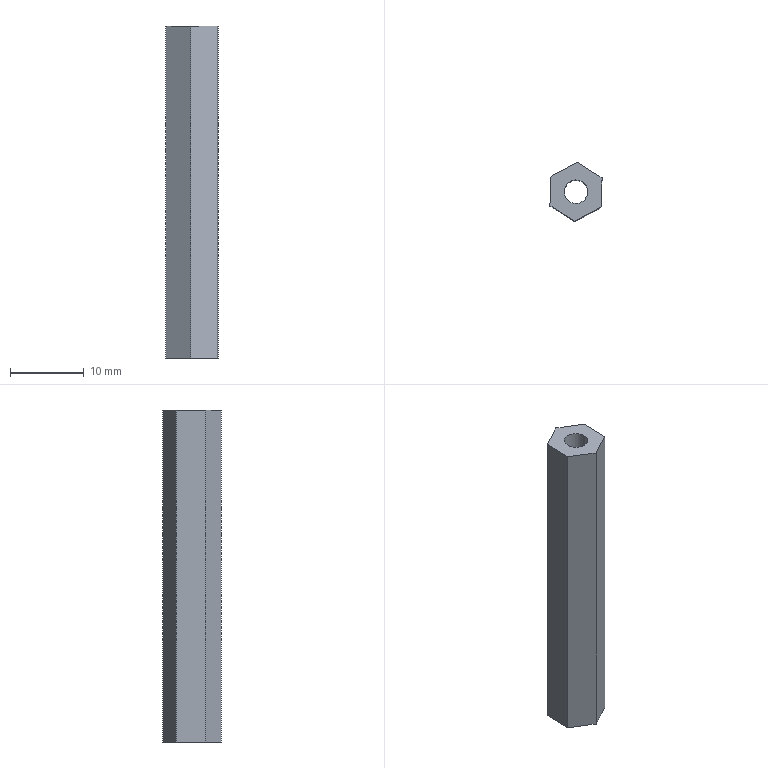Component | SolidWorks | 25CopperPillar-Copy-1 | 1 solid | 10 faces | box 7.07 x 7.99 x 45 mm | volume 1509 mm3 | plane 8 | cylinder 2 | commonest cylinder face diameters 3.2 x2
STEP:
#1=CARTESIAN_POINT('',(1.915,2.002,1.929));
#2=VERTEX_POINT('',#1);
#3=CARTESIAN_POINT('',(2.022,1.935,1.929));
#4=VERTEX_POINT('',#3);
#5=CARTESIAN_POINT('',(1.969,1.969,1.929));
#6=DIRECTION('',(0.,0.,1.));
#7=DIRECTION('',(0.8471,-0.5314,0.));
#8=AXIS2_PLACEMENT_3D('',#5,#6,#7);
#9=CIRCLE('',#8,0.06299);
#10=EDGE_CURVE('',#2,#4,#9,.T.);
#11=ORIENTED_EDGE('',*,*,#10,.T.);
#12=CARTESIAN_POINT('',(2.022,1.935,0.1575));
#13=VERTEX_POINT('',#12);
#14=CARTESIAN_POINT('',(2.022,1.935,1.929));
#15=DIRECTION('',(0.,0.,-1.));
#16=VECTOR('',#15,39.37);
#17=LINE('',#14,#16);
#18=EDGE_CURVE('',#4,#13,#17,.T.);
#19=ORIENTED_EDGE('',*,*,#18,.T.);
#20=CARTESIAN_POINT('',(1.915,2.002,0.1575));
#21=VERTEX_POINT('',#20);
#22=CARTESIAN_POINT('',(1.969,1.969,0.1575));
#23=DIRECTION('',(0.,0.,1.));
#24=DIRECTION('',(0.8471,-0.5314,0.));
#25=AXIS2_PLACEMENT_3D('',#22,#23,#24);
#26=CIRCLE('',#25,0.06299);
#27=EDGE_CURVE('',#21,#13,#26,.T.);
#28=ORIENTED_EDGE('',*,*,#27,.F.);
#29=CARTESIAN_POINT('',(1.915,2.002,1.929));
#30=DIRECTION('',(0.,0.,-1.));
#31=VECTOR('',#30,39.37);
#32=LINE('',#29,#31);
#33=EDGE_CURVE('',#2,#21,#32,.T.);
#34=ORIENTED_EDGE('',*,*,#33,.F.);
#35=EDGE_LOOP('',(#11,#19,#28,#34));
#36=FACE_OUTER_BOUND('',#35,.T.);
#37=CARTESIAN_POINT('',(1.969,1.969,1.929));
#38=DIRECTION('',(0.,0.,-1.));
#39=DIRECTION('',(-0.8471,0.5314,0.));
#40=AXIS2_PLACEMENT_3D('',#37,#38,#39);
#41=CYLINDRICAL_SURFACE('',#40,0.06299);
#42=ADVANCED_FACE('',(#36),#41,.F.);
#43=CARTESIAN_POINT('',(1.963,1.811,1.929));
#44=VERTEX_POINT('',#43);
#45=CARTESIAN_POINT('',(2.102,1.885,1.929));
#46=VERTEX_POINT('',#45);
#47=CARTESIAN_POINT('',(1.963,1.811,1.929));
#48=DIRECTION('',(0.8838,0.4679,0.));
#49=VECTOR('',#48,39.37);
#50=LINE('',#47,#49);
#51=EDGE_CURVE('',#44,#46,#50,.T.);
#52=ORIENTED_EDGE('',*,*,#51,.T.);
#53=CARTESIAN_POINT('',(2.108,2.042,1.929));
#54=VERTEX_POINT('',#53);
#55=CARTESIAN_POINT('',(2.102,1.885,1.929));
#56=DIRECTION('',(0.03664,0.9993,0.));
#57=VECTOR('',#56,39.37);
#58=LINE('',#55,#57);
#59=EDGE_CURVE('',#46,#54,#58,.T.);
#60=ORIENTED_EDGE('',*,*,#59,.T.);
#61=CARTESIAN_POINT('',(1.974,2.126,1.929));
#62=VERTEX_POINT('',#61);
#63=CARTESIAN_POINT('',(2.108,2.042,1.929));
#64=DIRECTION('',(-0.8471,0.5314,0.));
#65=VECTOR('',#64,39.37);
#66=LINE('',#63,#65);
#67=EDGE_CURVE('',#54,#62,#66,.T.);
#68=ORIENTED_EDGE('',*,*,#67,.T.);
#69=CARTESIAN_POINT('',(1.835,2.052,1.929));
#70=VERTEX_POINT('',#69);
#71=CARTESIAN_POINT('',(1.974,2.126,1.929));
#72=DIRECTION('',(-0.8838,-0.4679,0.));
#73=VECTOR('',#72,39.37);
#74=LINE('',#71,#73);
#75=EDGE_CURVE('',#62,#70,#74,.T.);
#76=ORIENTED_EDGE('',*,*,#75,.T.);
#77=CARTESIAN_POINT('',(1.829,1.895,1.929));
#78=VERTEX_POINT('',#77);
#79=CARTESIAN_POINT('',(1.835,2.052,1.929));
#80=DIRECTION('',(-0.03664,-0.9993,0.));
#81=VECTOR('',#80,39.37);
#82=LINE('',#79,#81);
#83=EDGE_CURVE('',#70,#78,#82,.T.);
#84=ORIENTED_EDGE('',*,*,#83,.T.);
#85=CARTESIAN_POINT('',(1.829,1.895,1.929));
#86=DIRECTION('',(0.8471,-0.5314,0.));
#87=VECTOR('',#86,39.37);
#88=LINE('',#85,#87);
#89=EDGE_CURVE('',#78,#44,#88,.T.);
#90=ORIENTED_EDGE('',*,*,#89,.T.);
#91=EDGE_LOOP('',(#52,#60,#68,#76,#84,#90));
#92=FACE_OUTER_BOUND('',#91,.T.);
#93=ORIENTED_EDGE('',*,*,#10,.F.);
#94=CARTESIAN_POINT('',(1.969,1.969,1.929));
#95=DIRECTION('',(0.,0.,1.));
#96=DIRECTION('',(0.8471,-0.5314,0.));
#97=AXIS2_PLACEMENT_3D('',#94,#95,#96);
#98=CIRCLE('',#97,0.06299);
#99=EDGE_CURVE('',#4,#2,#98,.T.);
#100=ORIENTED_EDGE('',*,*,#99,.F.);
#101=EDGE_LOOP('',(#93,#100));
#102=FACE_BOUND('',#101,.T.);
#103=CARTESIAN_POINT('',(1.969,1.969,1.929));
#104=DIRECTION('',(0.,0.,1.));
#105=DIRECTION('',(0.8471,-0.5314,0.));
#106=AXIS2_PLACEMENT_3D('',#103,#104,#105);
#107=PLANE('',#106);
#108=ADVANCED_FACE('',(#92,#102),#107,.T.);
#109=CARTESIAN_POINT('',(1.963,1.811,0.1575));
#110=VERTEX_POINT('',#109);
#111=CARTESIAN_POINT('',(2.102,1.885,0.1575));
#112=VERTEX_POINT('',#111);
#113=CARTESIAN_POINT('',(1.963,1.811,0.1575));
#114=DIRECTION('',(0.8838,0.4679,0.));
#115=VECTOR('',#114,39.37);
#116=LINE('',#113,#115);
#117=EDGE_CURVE('',#110,#112,#116,.T.);
#118=ORIENTED_EDGE('',*,*,#117,.F.);
#119=CARTESIAN_POINT('',(1.829,1.895,0.1575));
#120=VERTEX_POINT('',#119);
#121=CARTESIAN_POINT('',(1.829,1.895,0.1575));
#122=DIRECTION('',(0.8471,-0.5314,0.));
#123=VECTOR('',#122,39.37);
#124=LINE('',#121,#123);
#125=EDGE_CURVE('',#120,#110,#124,.T.);
#126=ORIENTED_EDGE('',*,*,#125,.F.);
#127=CARTESIAN_POINT('',(1.835,2.052,0.1575));
#128=VERTEX_POINT('',#127);
#129=CARTESIAN_POINT('',(1.835,2.052,0.1575));
#130=DIRECTION('',(-0.03664,-0.9993,0.));
#131=VECTOR('',#130,39.37);
#132=LINE('',#129,#131);
#133=EDGE_CURVE('',#128,#120,#132,.T.);
#134=ORIENTED_EDGE('',*,*,#133,.F.);
#135=CARTESIAN_POINT('',(1.974,2.126,0.1575));
#136=VERTEX_POINT('',#135);
#137=CARTESIAN_POINT('',(1.974,2.126,0.1575));
#138=DIRECTION('',(-0.8838,-0.4679,0.));
#139=VECTOR('',#138,39.37);
#140=LINE('',#137,#139);
#141=EDGE_CURVE('',#136,#128,#140,.T.);
#142=ORIENTED_EDGE('',*,*,#141,.F.);
#143=CARTESIAN_POINT('',(2.108,2.042,0.1575));
#144=VERTEX_POINT('',#143);
#145=CARTESIAN_POINT('',(2.108,2.042,0.1575));
#146=DIRECTION('',(-0.8471,0.5314,0.));
#147=VECTOR('',#146,39.37);
#148=LINE('',#145,#147);
#149=EDGE_CURVE('',#144,#136,#148,.T.);
#150=ORIENTED_EDGE('',*,*,#149,.F.);
#151=CARTESIAN_POINT('',(2.102,1.885,0.1575));
#152=DIRECTION('',(0.03664,0.9993,0.));
#153=VECTOR('',#152,39.37);
#154=LINE('',#151,#153);
#155=EDGE_CURVE('',#112,#144,#154,.T.);
#156=ORIENTED_EDGE('',*,*,#155,.F.);
#157=EDGE_LOOP('',(#118,#126,#134,#142,#150,#156));
#158=FACE_OUTER_BOUND('',#157,.T.);
#159=ORIENTED_EDGE('',*,*,#27,.T.);
#160=CARTESIAN_POINT('',(1.969,1.969,0.1575));
#161=DIRECTION('',(0.,0.,1.));
#162=DIRECTION('',(0.8471,-0.5314,0.));
#163=AXIS2_PLACEMENT_3D('',#160,#161,#162);
#164=CIRCLE('',#163,0.06299);
#165=EDGE_CURVE('',#13,#21,#164,.T.);
#166=ORIENTED_EDGE('',*,*,#165,.T.);
#167=EDGE_LOOP('',(#159,#166));
#168=FACE_BOUND('',#167,.T.);
#169=CARTESIAN_POINT('',(1.969,1.969,0.1575));
#170=DIRECTION('',(0.,0.,1.));
#171=DIRECTION('',(0.8471,-0.5314,0.));
#172=AXIS2_PLACEMENT_3D('',#169,#170,#171);
#173=PLANE('',#172);
#174=ADVANCED_FACE('',(#158,#168),#173,.F.);
#175=ORIENTED_EDGE('',*,*,#117,.T.);
#176=CARTESIAN_POINT('',(2.102,1.885,1.929));
#177=DIRECTION('',(0.,0.,-1.));
#178=VECTOR('',#177,39.37);
#179=LINE('',#176,#178);
#180=EDGE_CURVE('',#46,#112,#179,.T.);
#181=ORIENTED_EDGE('',*,*,#180,.F.);
#182=ORIENTED_EDGE('',*,*,#51,.F.);
#183=CARTESIAN_POINT('',(1.963,1.811,1.929));
#184=DIRECTION('',(0.,0.,-1.));
#185=VECTOR('',#184,39.37);
#186=LINE('',#183,#185);
#187=EDGE_CURVE('',#44,#110,#186,.T.);
#188=ORIENTED_EDGE('',*,*,#187,.T.);
#189=EDGE_LOOP('',(#175,#181,#182,#188));
#190=FACE_OUTER_BOUND('',#189,.T.);
#191=CARTESIAN_POINT('',(1.963,1.811,1.929));
#192=DIRECTION('',(-0.4679,0.8838,0.));
#193=DIRECTION('',(-0.8838,-0.4679,0.));
#194=AXIS2_PLACEMENT_3D('',#191,#192,#193);
#195=PLANE('',#194);
#196=ADVANCED_FACE('',(#190),#195,.F.);
#197=ORIENTED_EDGE('',*,*,#155,.T.);
#198=CARTESIAN_POINT('',(2.108,2.042,1.929));
#199=DIRECTION('',(0.,0.,-1.));
#200=VECTOR('',#199,39.37);
#201=LINE('',#198,#200);
#202=EDGE_CURVE('',#54,#144,#201,.T.);
#203=ORIENTED_EDGE('',*,*,#202,.F.);
#204=ORIENTED_EDGE('',*,*,#59,.F.);
#205=ORIENTED_EDGE('',*,*,#180,.T.);
#206=EDGE_LOOP('',(#197,#203,#204,#205));
#207=FACE_OUTER_BOUND('',#206,.T.);
#208=CARTESIAN_POINT('',(2.102,1.885,1.929));
#209=DIRECTION('',(-0.9993,0.03664,0.));
#210=DIRECTION('',(-0.03664,-0.9993,0.));
#211=AXIS2_PLACEMENT_3D('',#208,#209,#210);
#212=PLANE('',#211);
#213=ADVANCED_FACE('',(#207),#212,.F.);
#214=ORIENTED_EDGE('',*,*,#149,.T.);
#215=CARTESIAN_POINT('',(1.974,2.126,1.929));
#216=DIRECTION('',(0.,0.,-1.));
#217=VECTOR('',#216,39.37);
#218=LINE('',#215,#217);
#219=EDGE_CURVE('',#62,#136,#218,.T.);
#220=ORIENTED_EDGE('',*,*,#219,.F.);
#221=ORIENTED_EDGE('',*,*,#67,.F.);
#222=ORIENTED_EDGE('',*,*,#202,.T.);
#223=EDGE_LOOP('',(#214,#220,#221,#222));
#224=FACE_OUTER_BOUND('',#223,.T.);
#225=CARTESIAN_POINT('',(2.108,2.042,1.929));
#226=DIRECTION('',(-0.5314,-0.8471,0.));
#227=DIRECTION('',(0.8471,-0.5314,0.));
#228=AXIS2_PLACEMENT_3D('',#225,#226,#227);
#229=PLANE('',#228);
#230=ADVANCED_FACE('',(#224),#229,.F.);
#231=ORIENTED_EDGE('',*,*,#141,.T.);
#232=CARTESIAN_POINT('',(1.835,2.052,1.929));
#233=DIRECTION('',(0.,0.,-1.));
#234=VECTOR('',#233,39.37);
#235=LINE('',#232,#234);
#236=EDGE_CURVE('',#70,#128,#235,.T.);
#237=ORIENTED_EDGE('',*,*,#236,.F.);
#238=ORIENTED_EDGE('',*,*,#75,.F.);
#239=ORIENTED_EDGE('',*,*,#219,.T.);
#240=EDGE_LOOP('',(#231,#237,#238,#239));
#241=FACE_OUTER_BOUND('',#240,.T.);
#242=CARTESIAN_POINT('',(1.974,2.126,1.929));
#243=DIRECTION('',(0.4679,-0.8838,0.));
#244=DIRECTION('',(0.8838,0.4679,0.));
#245=AXIS2_PLACEMENT_3D('',#242,#243,#244);
#246=PLANE('',#245);
#247=ADVANCED_FACE('',(#241),#246,.F.);
#248=ORIENTED_EDGE('',*,*,#133,.T.);
#249=CARTESIAN_POINT('',(1.829,1.895,1.929));
#250=DIRECTION('',(0.,0.,-1.));
#251=VECTOR('',#250,39.37);
#252=LINE('',#249,#251);
#253=EDGE_CURVE('',#78,#120,#252,.T.);
#254=ORIENTED_EDGE('',*,*,#253,.F.);
#255=ORIENTED_EDGE('',*,*,#83,.F.);
#256=ORIENTED_EDGE('',*,*,#236,.T.);
#257=EDGE_LOOP('',(#248,#254,#255,#256));
#258=FACE_OUTER_BOUND('',#257,.T.);
#259=CARTESIAN_POINT('',(1.835,2.052,1.929));
#260=DIRECTION('',(0.9993,-0.03664,0.));
#261=DIRECTION('',(0.03664,0.9993,0.));
#262=AXIS2_PLACEMENT_3D('',#259,#260,#261);
#263=PLANE('',#262);
#264=ADVANCED_FACE('',(#258),#263,.F.);
#265=ORIENTED_EDGE('',*,*,#125,.T.);
#266=ORIENTED_EDGE('',*,*,#187,.F.);
#267=ORIENTED_EDGE('',*,*,#89,.F.);
#268=ORIENTED_EDGE('',*,*,#253,.T.);
#269=EDGE_LOOP('',(#265,#266,#267,#268));
#270=FACE_OUTER_BOUND('',#269,.T.);
#271=CARTESIAN_POINT('',(1.829,1.895,1.929));
#272=DIRECTION('',(0.5314,0.8471,0.));
#273=DIRECTION('',(-0.8471,0.5314,0.));
#274=AXIS2_PLACEMENT_3D('',#271,#272,#273);
#275=PLANE('',#274);
#276=ADVANCED_FACE('',(#270),#275,.F.);
#277=ORIENTED_EDGE('',*,*,#18,.F.);
#278=ORIENTED_EDGE('',*,*,#99,.T.);
#279=ORIENTED_EDGE('',*,*,#33,.T.);
#280=ORIENTED_EDGE('',*,*,#165,.F.);
#281=EDGE_LOOP('',(#277,#278,#279,#280));
#282=FACE_OUTER_BOUND('',#281,.T.);
#283=CARTESIAN_POINT('',(1.969,1.969,1.929));
#284=DIRECTION('',(0.,0.,-1.));
#285=DIRECTION('',(-0.8471,0.5314,0.));
#286=AXIS2_PLACEMENT_3D('',#283,#284,#285);
#287=CYLINDRICAL_SURFACE('',#286,0.06299);
#288=ADVANCED_FACE('',(#282),#287,.F.);
#289=CLOSED_SHELL('',(#42,#108,#174,#196,#213,#230,#247,#264,#276,#288));
#290=MANIFOLD_SOLID_BREP('',#289);
#291=CARTESIAN_POINT('',(0.,0.,0.));
#292=DIRECTION('',(0.,0.,1.));
#293=DIRECTION('',(1.,0.,0.));
#294=AXIS2_PLACEMENT_3D('',#291,#292,#293);
#295=(LENGTH_UNIT()NAMED_UNIT(*)SI_UNIT($,.METRE.));
#296=LENGTH_MEASURE_WITH_UNIT(LENGTH_MEASURE(0.0254),#295);
#297=DIMENSIONAL_EXPONENTS(1.,0.,0.,0.,0.,0.,0.);
#298=(CONVERSION_BASED_UNIT('',#296)LENGTH_UNIT()NAMED_UNIT(#297));
#299=UNCERTAINTY_MEASURE_WITH_UNIT(LENGTH_MEASURE(0.00001),#298,'','');
#300=(NAMED_UNIT(*)PLANE_ANGLE_UNIT()SI_UNIT($,.RADIAN.));
#301=(NAMED_UNIT(*)SI_UNIT($,.STERADIAN.)SOLID_ANGLE_UNIT());
#302=(GEOMETRIC_REPRESENTATION_CONTEXT(3)GLOBAL_UNCERTAINTY_ASSIGNED_CONTEXT((#299))GLOBAL_UNIT_ASSIGNED_CONTEXT((#298,#300,#301))REPRESENTATION_CONTEXT('',''));
#303=ADVANCED_BREP_SHAPE_REPRESENTATION('',(#290,#294),#302);
#304=COLOUR_RGB('',0.7922,0.8196,0.9333);
#305=FILL_AREA_STYLE_COLOUR('',#304);
#306=FILL_AREA_STYLE('',(#305));
#307=SURFACE_STYLE_FILL_AREA(#306);
#308=SURFACE_SIDE_STYLE('',(#307));
#309=SURFACE_STYLE_USAGE(.BOTH.,#308);
#310=PRESENTATION_STYLE_ASSIGNMENT((#309));
#311=STYLED_ITEM('',(#310),#290);
#312=(LENGTH_UNIT()NAMED_UNIT(*)SI_UNIT($,.METRE.));
#313=LENGTH_MEASURE_WITH_UNIT(LENGTH_MEASURE(0.0254),#312);
#314=DIMENSIONAL_EXPONENTS(1.,0.,0.,0.,0.,0.,0.);
#315=(CONVERSION_BASED_UNIT('',#313)LENGTH_UNIT()NAMED_UNIT(#314));
#316=UNCERTAINTY_MEASURE_WITH_UNIT(LENGTH_MEASURE(0.00001),#315,'','');
#317=(NAMED_UNIT(*)PLANE_ANGLE_UNIT()SI_UNIT($,.RADIAN.));
#318=(NAMED_UNIT(*)SI_UNIT($,.STERADIAN.)SOLID_ANGLE_UNIT());
#319=(GEOMETRIC_REPRESENTATION_CONTEXT(3)GLOBAL_UNCERTAINTY_ASSIGNED_CONTEXT((#316))GLOBAL_UNIT_ASSIGNED_CONTEXT((#315,#317,#318))REPRESENTATION_CONTEXT('',''));
#320=MECHANICAL_DESIGN_GEOMETRIC_PRESENTATION_REPRESENTATION('',(#311),#319);
#321=PRESENTATION_LAYER_ASSIGNMENT('','',(#311));